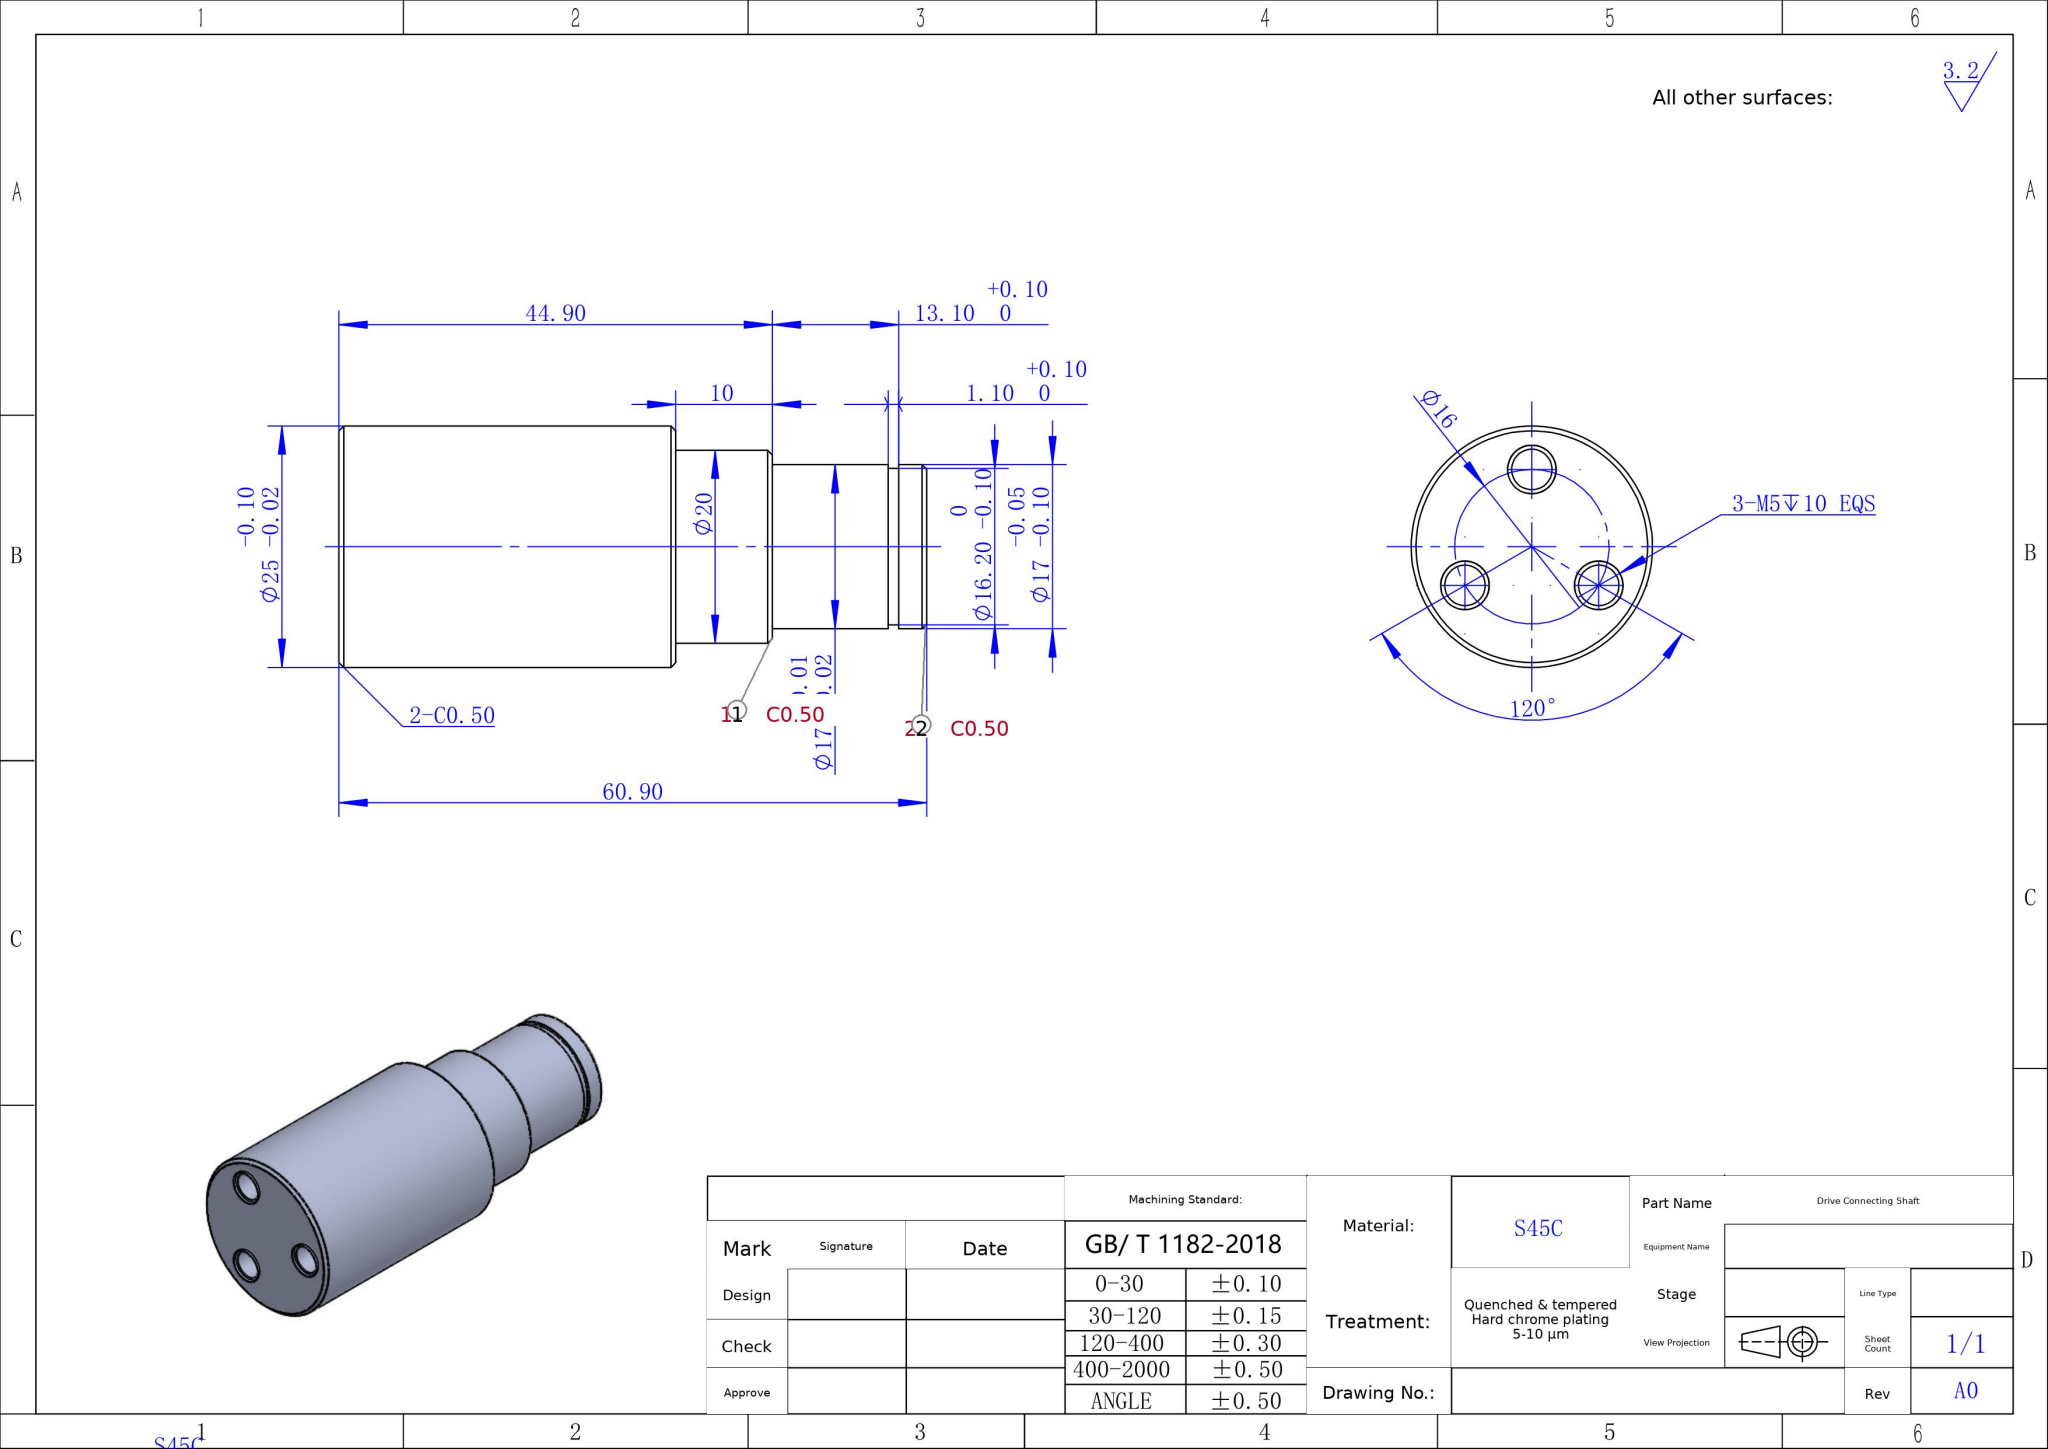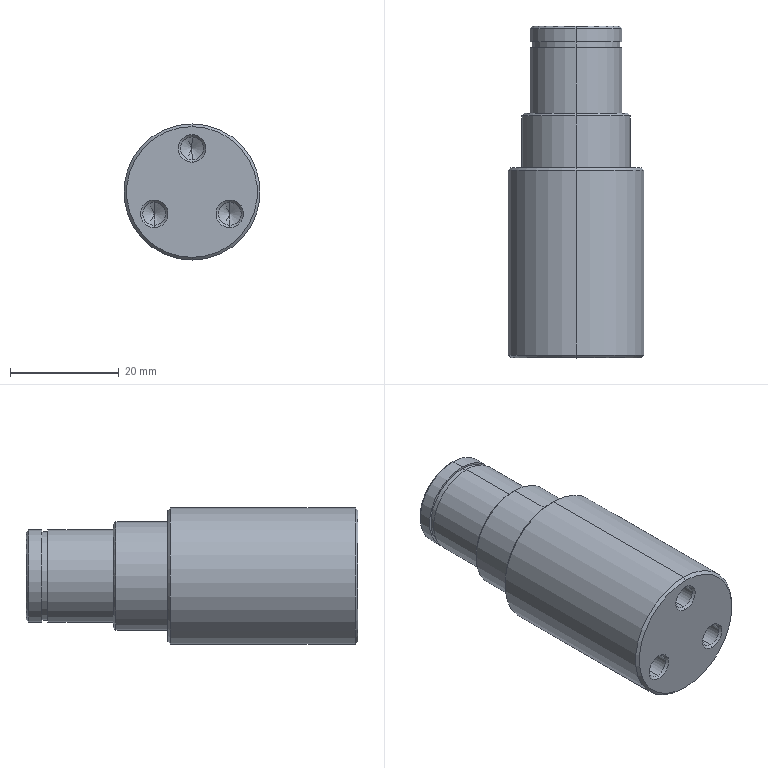Part | SolidWorks | mm | material S45C | 1 solid | 42 faces | box 25 x 60.9 x 25 mm | volume 23328 mm3 | cone 20 | cylinder 16 | plane 6 | commonest cylinder face diameters 4.2 x6 17 x4 25 x2 20 x2 16.2 x2
build123d program:
from build123d import *

# Parameters (mm, degrees)
CHAMFER1_SIZE              = 0.5
SKETCH5_R                  = 12.5
BOSS_EXTRUDE1_DEPTH        = 10
SKETCH6_R                  = 2.1
CUT_EXTRUDE1_DEPTH         = 10
M5_TAPPED_HOLE2_AT_2_COUNT = 2
M5_TAPPED_HOLE2_AT_2_PITCH = 13.856
M5_TAPPED_HOLE2_AT_3_COUNT = 2
M5_TAPPED_HOLE2_AT_3_PITCH = 13.856
CIRPATTERN1_COUNT          = 3


with BuildPart() as part:
    # Sketch1 → Revolve1 (revolve)
    with BuildSketch(Plane.XY, mode=Mode.PRIVATE) as revolve1_sk:
        Polygon((0, 0), (8.5, 0), (8.5, -2.9), (8.1, -2.9), (8.1, -4), (8.5, -4), (8.5, -16), (10, -16), (10, -26), (12.5, -26), (12.5, -60.9), (0, -60.9), align=None)
    revolve(revolve1_sk.sketch.rotate(Axis((0, 0, 0), (0, 1, 0)), 90), axis=Axis((0, 0, 0), (0, 1, 0)))

    # Chamfer1
    chamfer1_edges = [part.edges().sort_by_distance(p)[0] for p in [
        (0, -26, 12.5),
        (0, -16, 10),
        (0, 0, 8.5),
        (0, -60.9, 12.5),
    ]]
    chamfer(chamfer1_edges, length=CHAMFER1_SIZE)

    # Sketch10 → M5 Tapped Hole2 (revolve, cut)
    with BuildSketch(Plane(origin=(-6.928, -60.9, -4), x_dir=(0, 0, -1), z_dir=(1, 0, 0))):
        Polygon((0, 0), (0, 13.262), (2.1, 12), (2.1, 0.425), (2.525, 0), align=None)
    m5_tapped_hole2 = revolve(axis=Axis((-6.928, -67.25, -4), (0, 1, 0)), mode=Mode.SUBTRACT)

    # M5 Tapped Hole2 at 2: M5 Tapped Hole2 ×2
    with Locations(*[Vector(0.5, 0, 0.866) * (i * M5_TAPPED_HOLE2_AT_2_PITCH) for i in range(1, M5_TAPPED_HOLE2_AT_2_COUNT)]):
        add(m5_tapped_hole2, mode=Mode.SUBTRACT)

    # M5 Tapped Hole2 at 3: M5 Tapped Hole2 ×2
    with Locations(*[(i * M5_TAPPED_HOLE2_AT_3_PITCH, 0, 0) for i in range(1, M5_TAPPED_HOLE2_AT_3_COUNT)]):
        add(m5_tapped_hole2, mode=Mode.SUBTRACT)

    # CirPattern1: part ×3 about axis
    cirpattern1_axis = Axis((0, 0, 0), (0, -1, 0))


with BuildPart() as body_2:
    # Sketch5 → Boss-Extrude1 (new body)
    with BuildSketch(Plane.XZ.offset(60.9)):
        with Locations(Location((-44.263, 0, 0), (0, 0, 270))):
            Circle(SKETCH5_R)
    extrude(amount=BOSS_EXTRUDE1_DEPTH)

    # Sketch6 → Cut-Extrude1 (cut)
    with BuildSketch(Plane.XZ.offset(70.9)):
        with Locations(Location((-44.263, 7.5, 0), (0, 0, 270))):
            Circle(SKETCH6_R)
        with Locations(Location((-51.163, -4.451, 0), (0, 0, 270))):
            Circle(SKETCH6_R)
        with Locations(Location((-37.363, -4.451, 0), (0, 0, 90))):
            Circle(SKETCH6_R)
    extrude(amount=-CUT_EXTRUDE1_DEPTH, mode=Mode.SUBTRACT)


with BuildPart() as part_1:
    add(part.part)
    for i in range(1, CIRPATTERN1_COUNT):
        add(part.part.rotate(cirpattern1_axis, i * 360 / CIRPATTERN1_COUNT))


solid = part_1.part